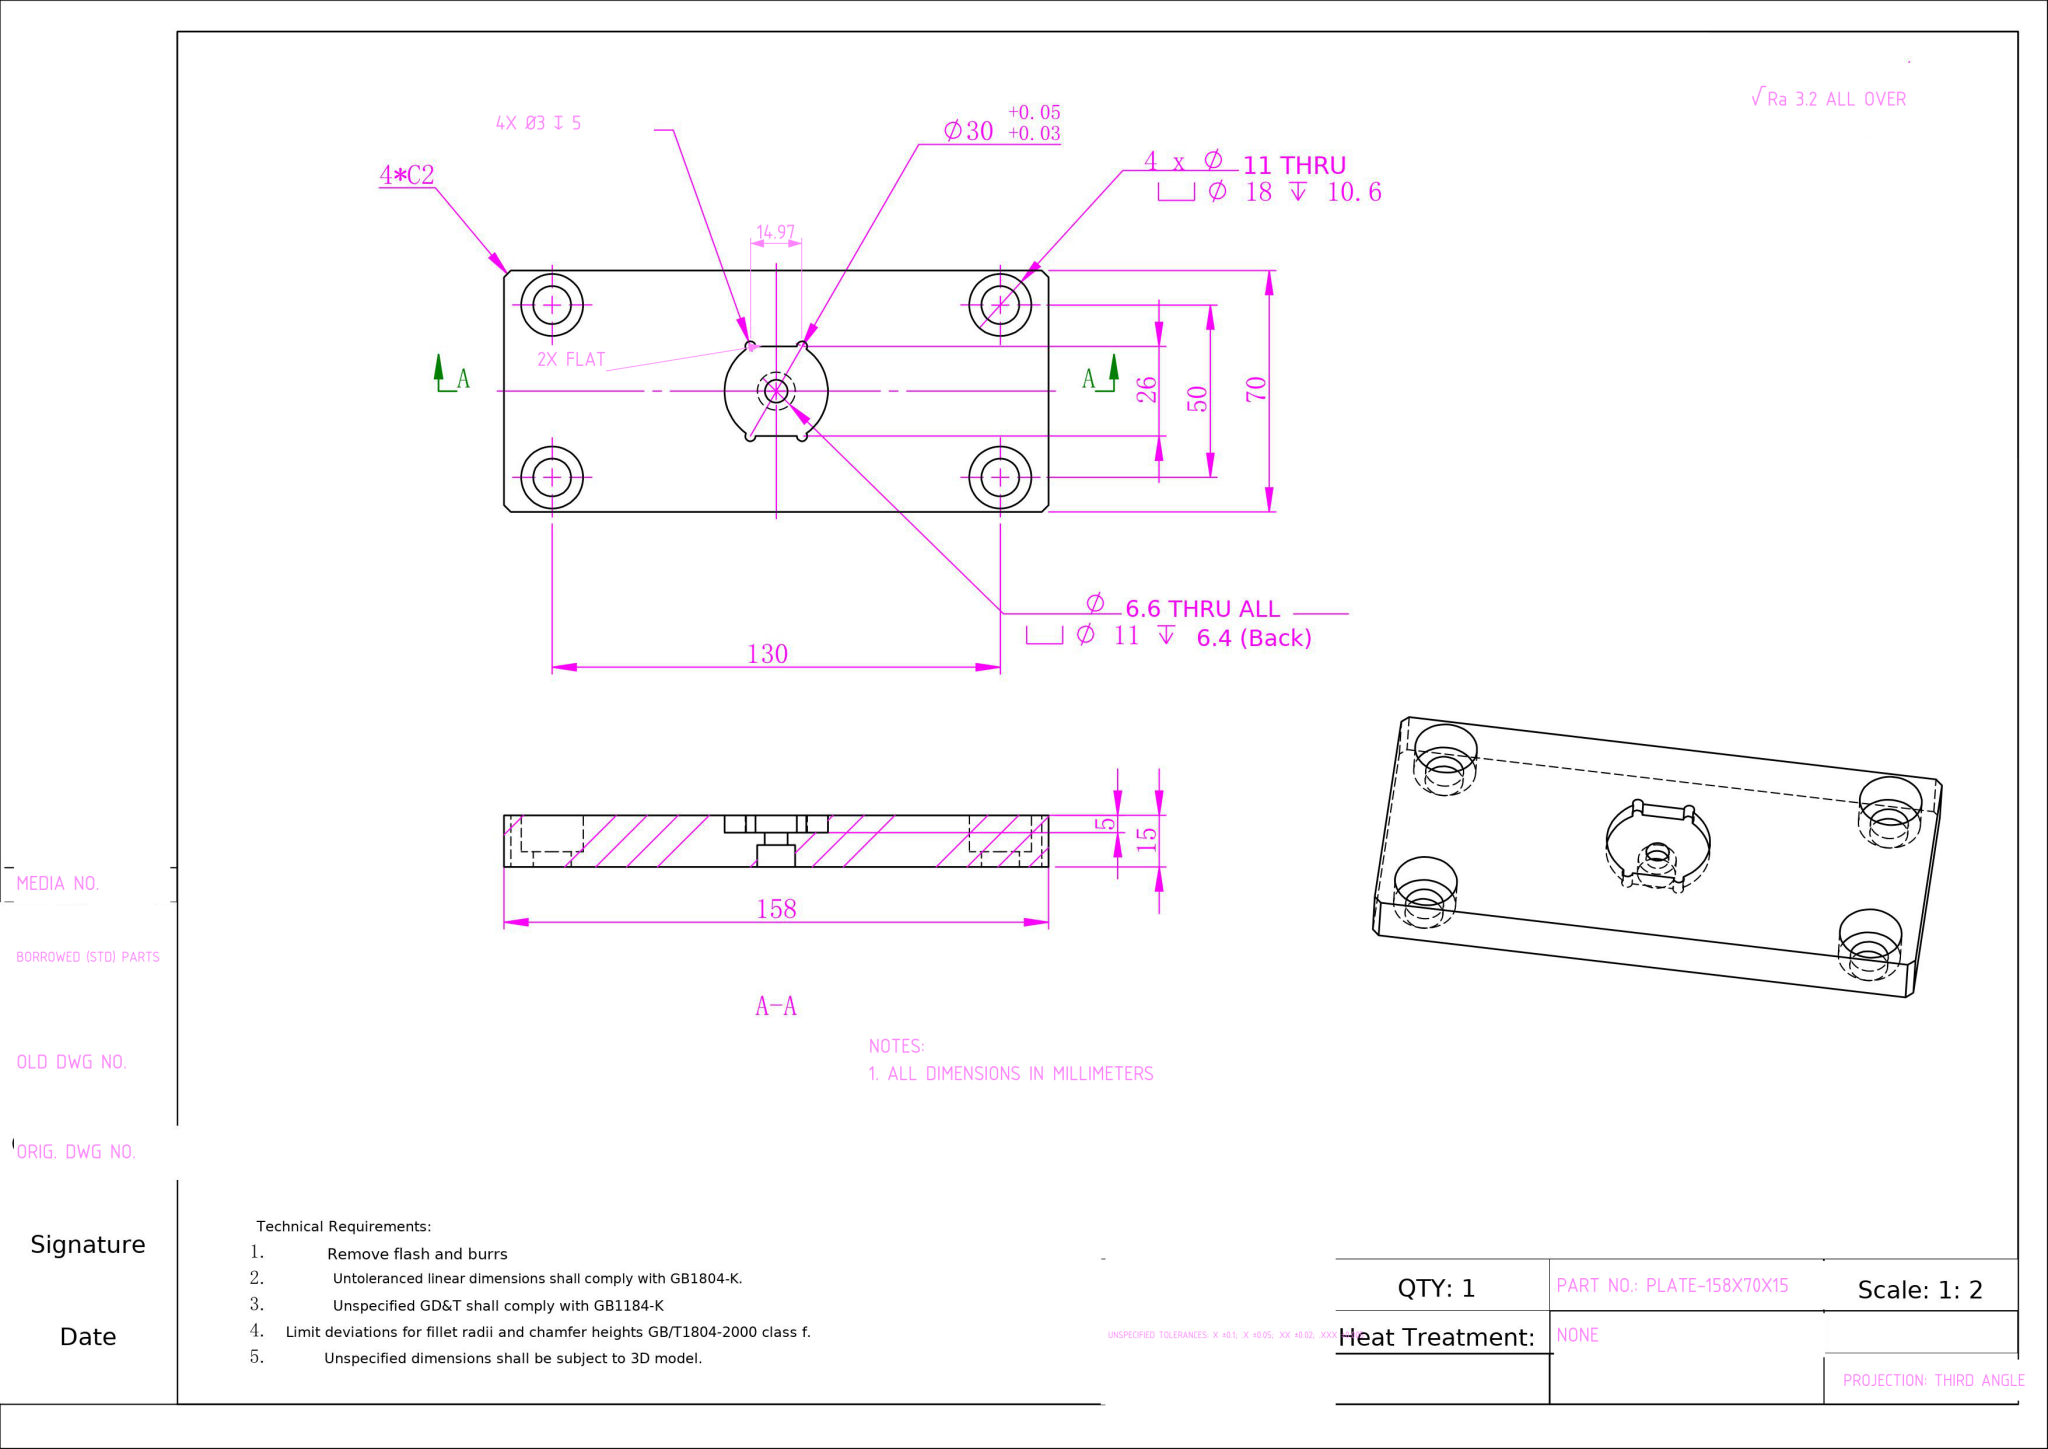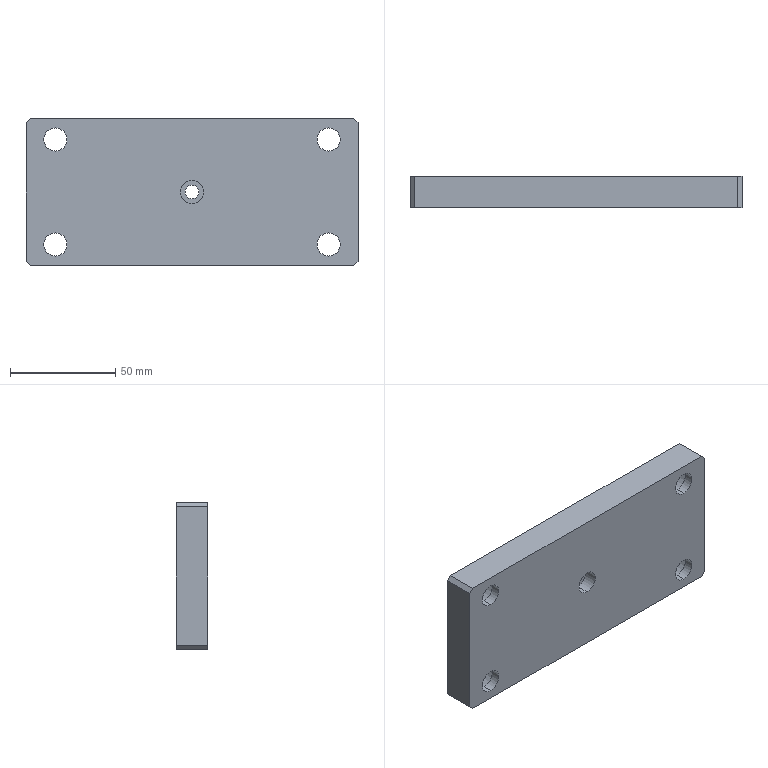Part | NX | mm | 1 solid | 46 faces | box 158 x 15 x 70 mm | volume 149171 mm3 | cylinder 28 | plane 18 | commonest cylinder face diameters 11 x10 18 x8 3 x6 6.6 x2 30 x2